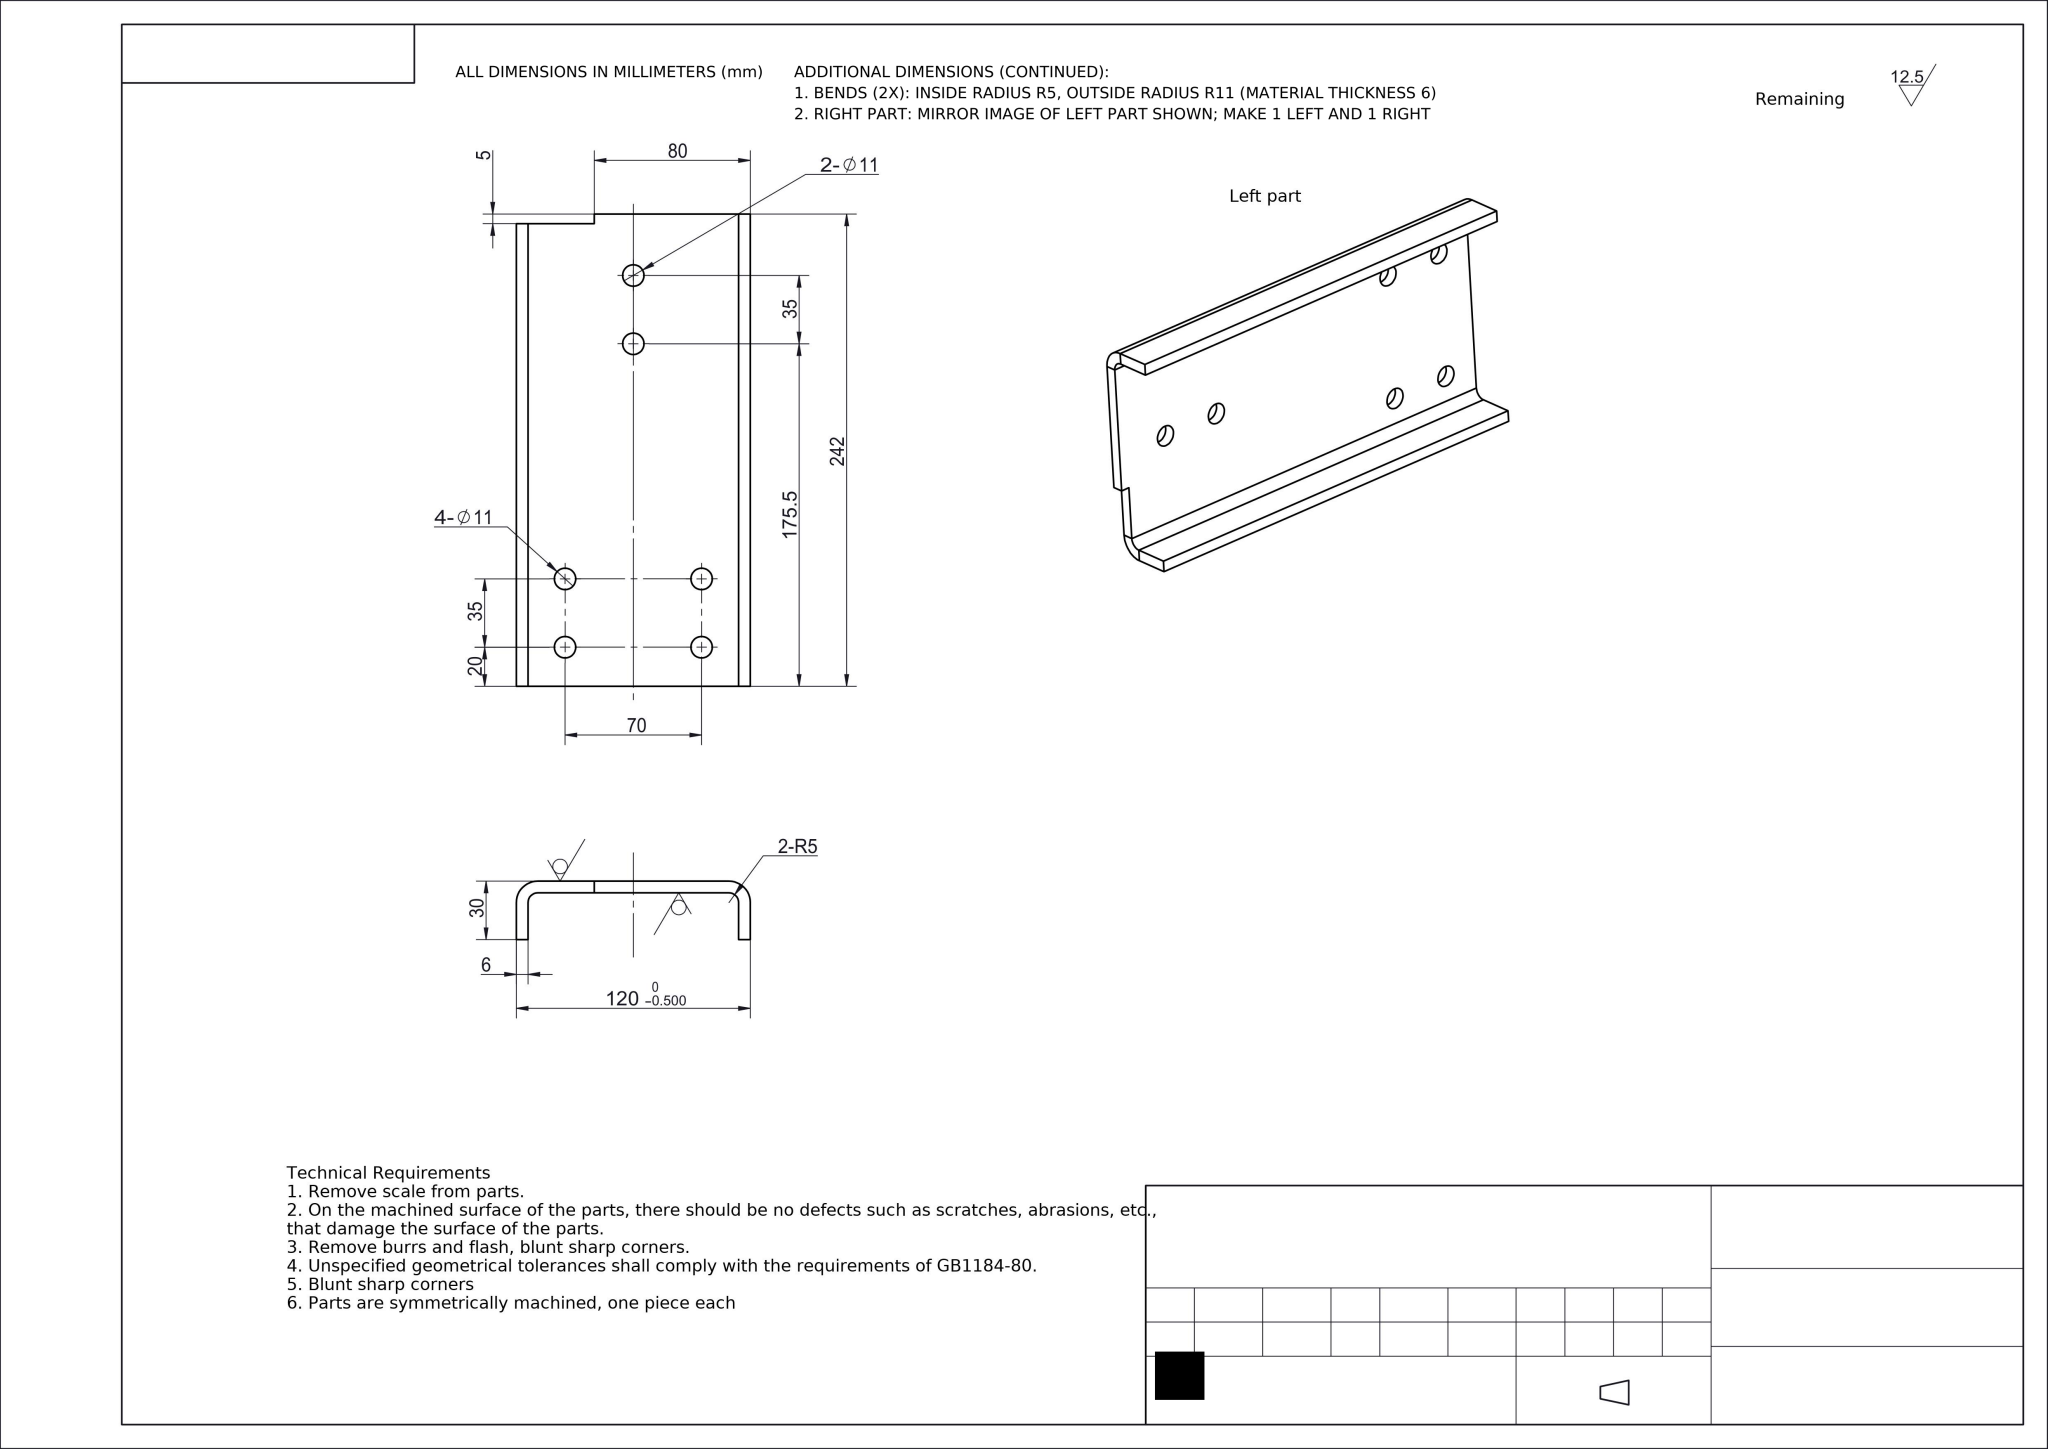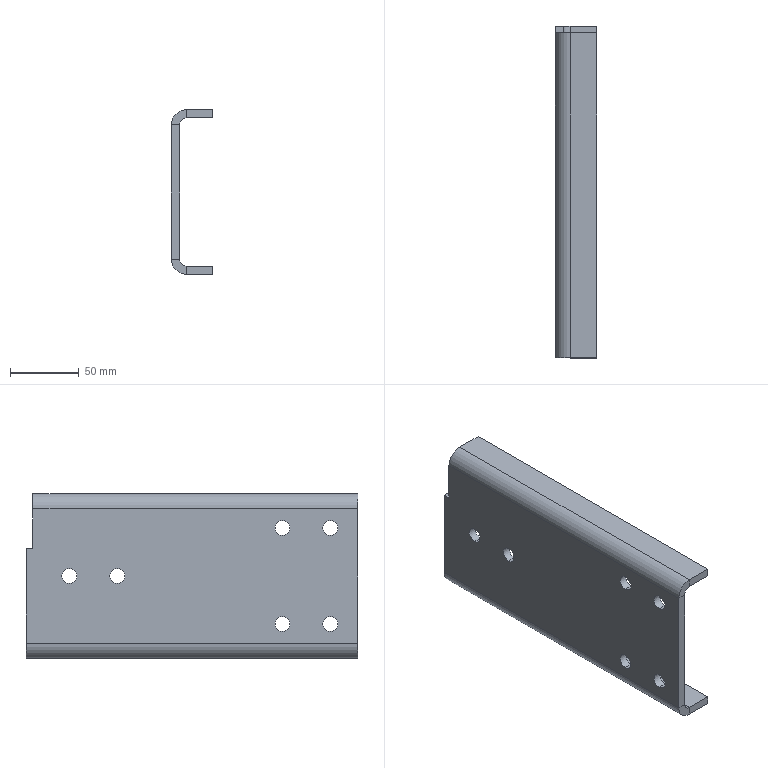Part | NX | mm | 1 solid | 36 faces | box 30 x 242 x 120 mm | volume 228727 mm3 | plane 20 | cylinder 16 | commonest cylinder face diameters 11 x12 10 x2 22 x2